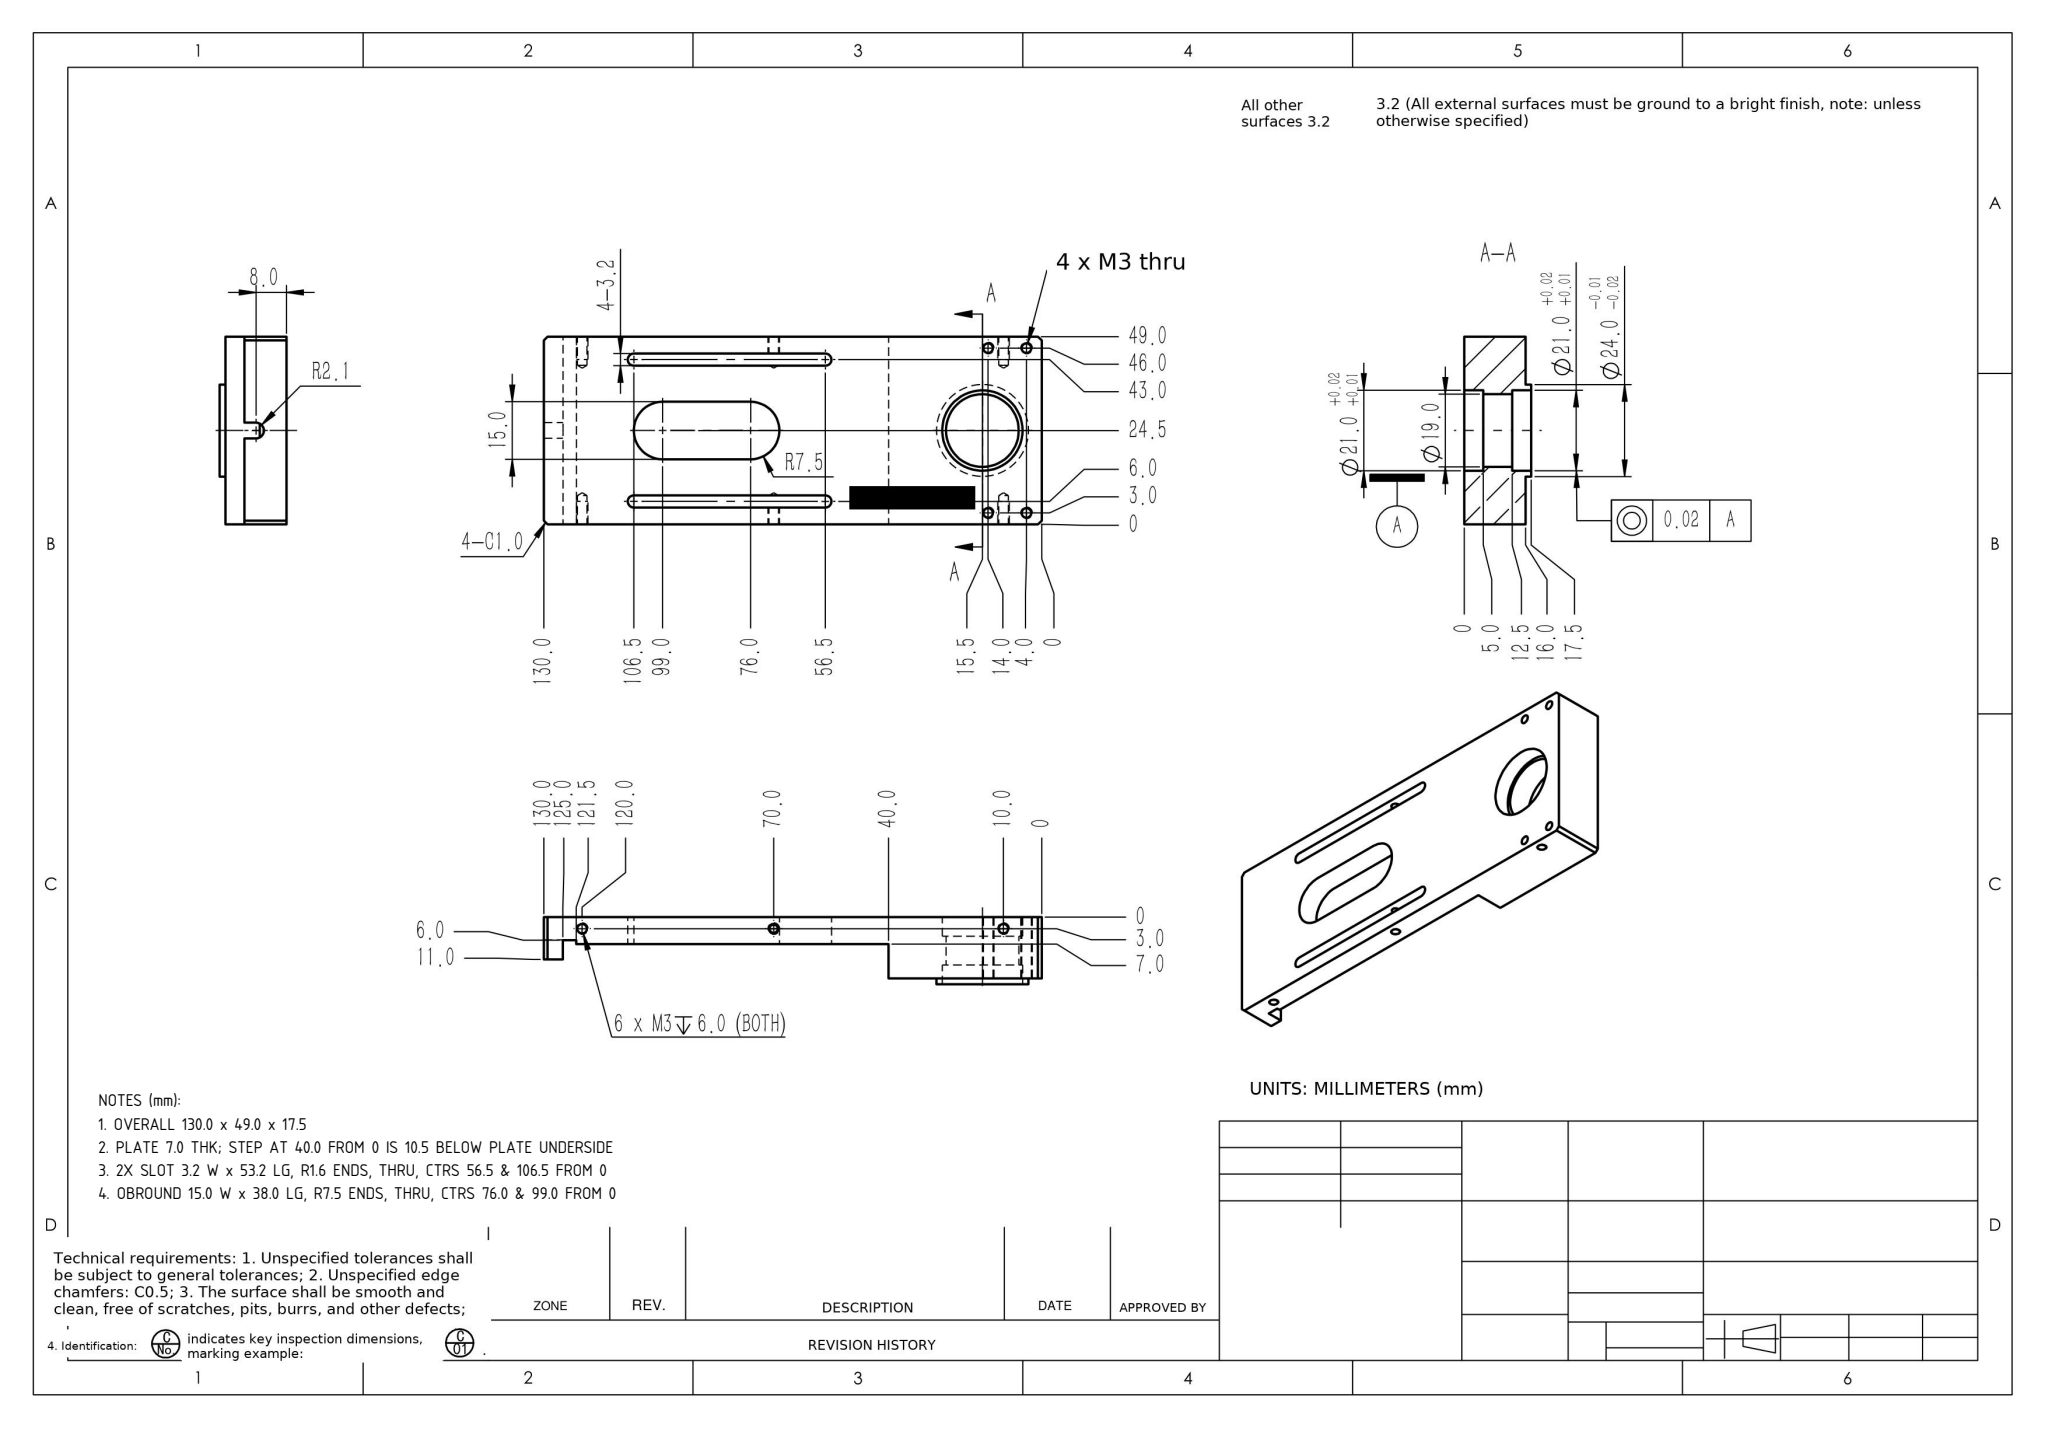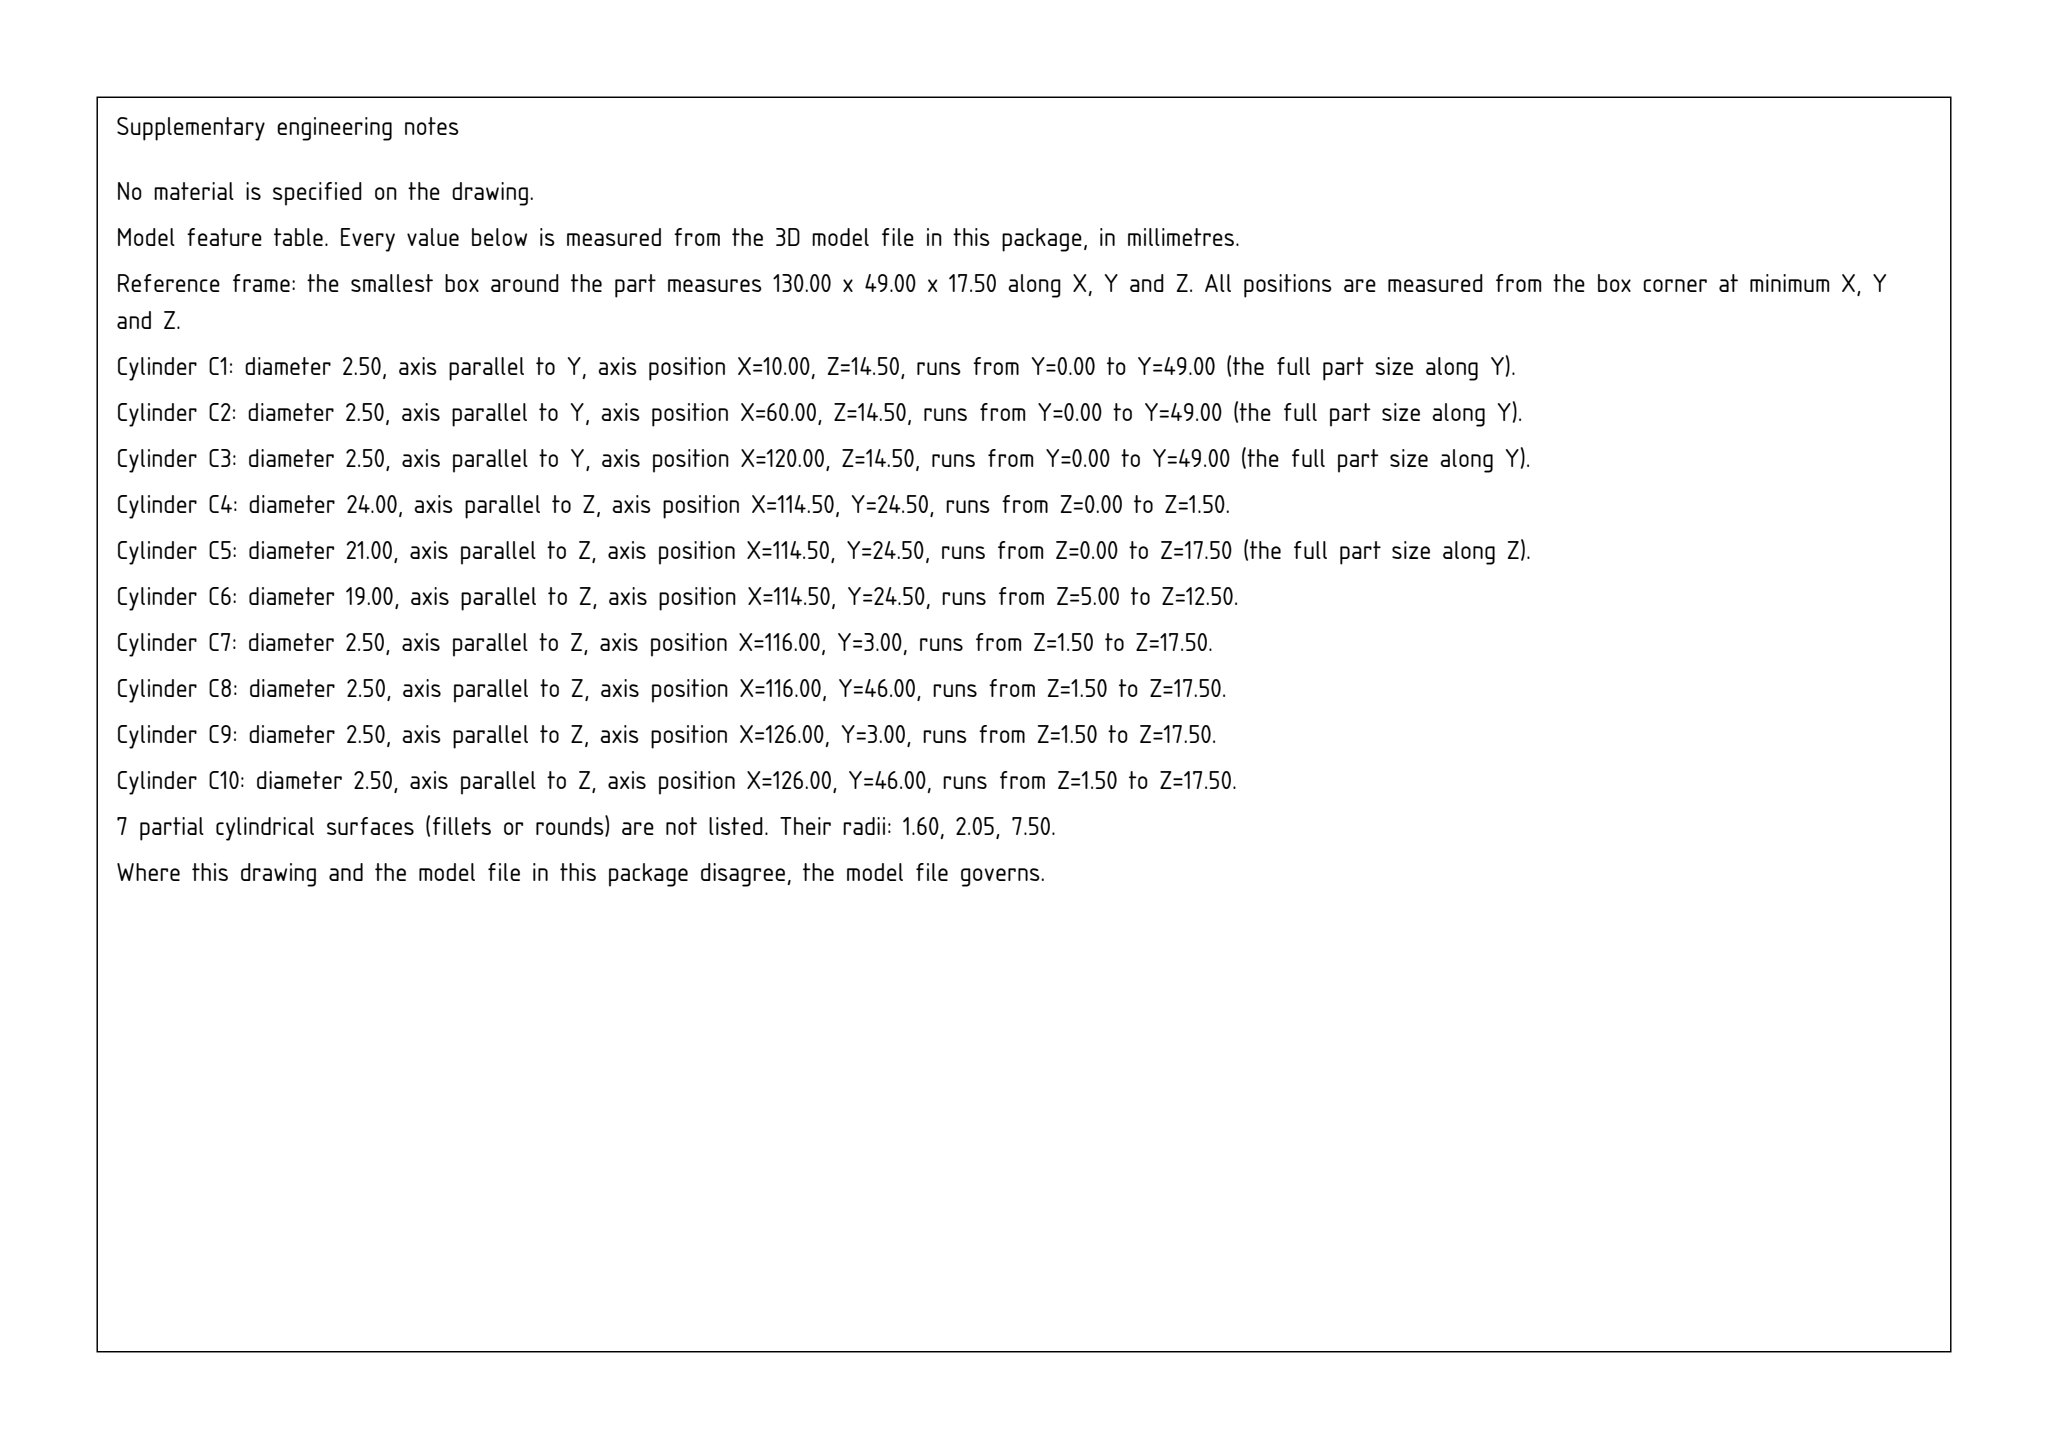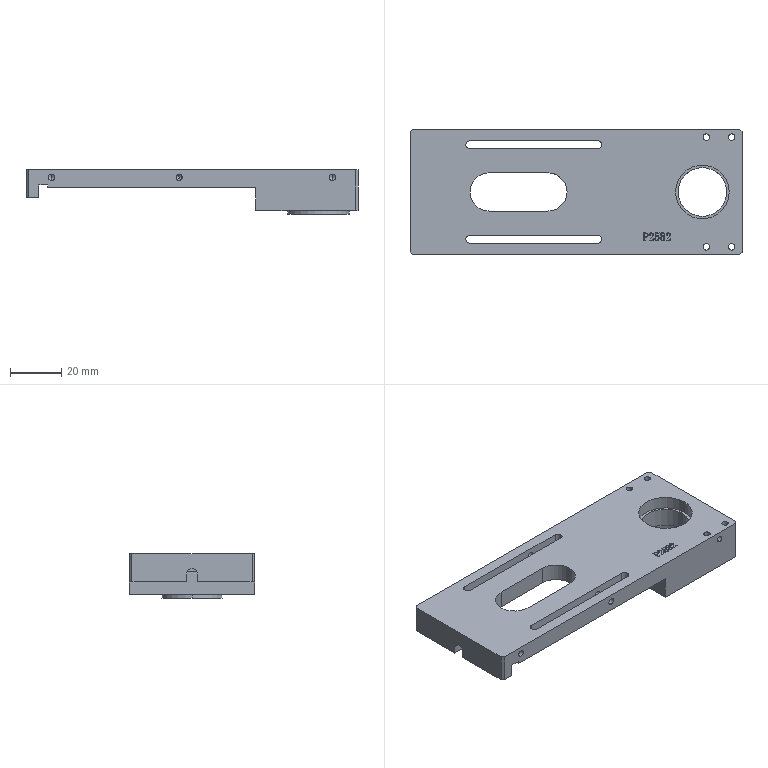Part | SolidWorks | mm | 1 solid | 89 faces | box 130 x 49 x 17.5 mm | volume 51490 mm3 | cylinder 39 | plane 38 | cone 12 | commonest cylinder face diameters 2.5 x20 3.2 x6 21 x4 15 x3 4.1 x2 24 x2 19 x2
Drawing notes:
OVERALL 130.0 x 49.0 x 17.5 | from the solid: bbox_xyz [130.0, 49.0, 17.5]
PLATE 7.0 THK; STEP AT 40.0 FROM 0 IS 10.5 BELOW PLATE UNDERSIDE | from the solid: z-cyl len 7.0 (z 10.5-17.5); x plane at 90.0 = 40.0 from RH end; boss z 0-17.5 vs plate btm z=10.5
2X SLOT 3.2 W x 53.2 LG, R1.6 ENDS, THRU, CTRS 56.5 & 106.5 FROM 0 | from the solid: Ø3.2 z-cyls at x=23.5 & 73.5, y=6.0 & 43.0, len 7.0 -> 50.0 btwn ctrs, 53.2 OAL, R1.6
OBROUND 15.0 W x 38.0 LG, R7.5 ENDS, THRU, CTRS 76.0 & 99.0 FROM 0 | from the solid: Ø15.0 z-cyls at x=31.0 & 54.0, y=24.5; y planes 17.0/32.0 = 15.0 W; 54-31+15=38.0 OAL